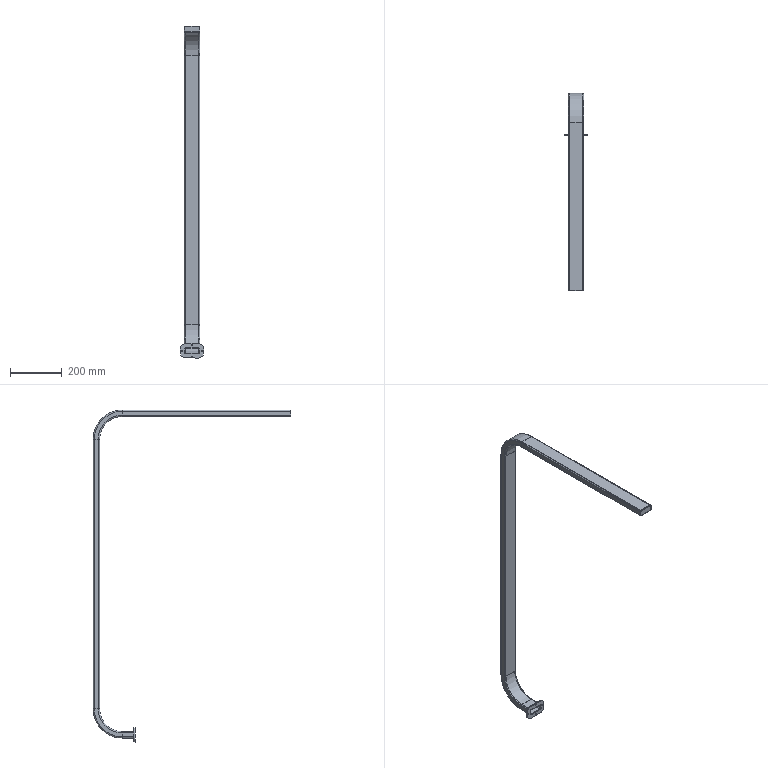Component | SolidWorks | HeightMeasurement-1 | 1 solid | 130 faces | box 90 x 762.5 x 1280 mm | volume 652548 mm3 | cylinder 58 | plane 44 | torus 28 | commonest cylinder face diameters 10 x12 6 x12 5 x8 2 x8 4 x4 40 x4 38.4 x2 225 x2
build123d program:
from build123d import *

# Parameters (mm, degrees)
BOSS_EXTRUDE1_START = -2
BOSS_EXTRUDE1_DEPTH = 2
FILLET1_R           = 2
BOSS_EXTRUDE2_DEPTH = 5
SKETCH6_R           = 2.5
CUT_EXTRUDE1_DEPTH  = 4
CUT_EXTRUDE2_REACH  = 1471.169
SKETCH7_R           = 19.2
FILLET5_R           = 1


with BuildPart() as part:
    # Scan-Thin Part2: sweep along a path in Sketch1
    with BuildLine(Plane(origin=(0, 0, 0), x_dir=(0, 0, -1), z_dir=(1, 0, 0))) as scan_thin_part2_path:
        Line((0, 0), (650, 0))
        ThreePointArc((650, 0), (720.711, -29.289), (750, -100))
        Line((750, -100), (750, -1140))
        ThreePointArc((750, -1140), (720.711, -1210.711), (650, -1240))
        Line((650, -1240), (600, -1240))
    # Sketch3 → Scan-Thin Part2 (sweep)
    with BuildSketch(Plane.XY):
        with BuildLine():
            Line((-25, 12.5), (25, 12.5))
            ThreePointArc((25, 12.5), (28.536, 11.036), (30, 7.5))
            Line((30, 7.5), (30, -7.5))
            ThreePointArc((30, -7.5), (28.536, -11.036), (25, -12.5))
            Line((25, -12.5), (-25, -12.5))
            ThreePointArc((-25, -12.5), (-28.536, -11.036), (-30, -7.5))
            Line((-30, -7.5), (-30, 7.5))
            ThreePointArc((-30, 7.5), (-28.536, 11.036), (-25, 12.5))
        make_face()
        with BuildLine():
            Line((-25, 10.5), (25, 10.5))
            ThreePointArc((25, 10.5), (27.121, 9.621), (28, 7.5))
            Line((28, 7.5), (28, -7.5))
            ThreePointArc((28, -7.5), (27.121, -9.621), (25, -10.5))
            Line((25, -10.5), (-25, -10.5))
            ThreePointArc((-25, -10.5), (-27.121, -9.621), (-28, -7.5))
            Line((-28, -7.5), (-28, 7.5))
            ThreePointArc((-28, 7.5), (-27.121, 9.621), (-25, 10.5))
        make_face(mode=Mode.SUBTRACT)
    sweep(path=scan_thin_part2_path.line)

    # Sketch4 → Boss-Extrude1 (add)
    with BuildSketch(Plane.XY.offset(BOSS_EXTRUDE1_START)):
        with BuildLine():
            Line((28, -7.5), (28, 7.5))
            ThreePointArc((28, 7.5), (27.121, 9.621), (25, 10.5))
            Line((25, 10.5), (-25, 10.5))
            ThreePointArc((-25, 10.5), (-27.121, 9.621), (-28, 7.5))
            Line((-28, 7.5), (-28, -7.5))
            ThreePointArc((-28, -7.5), (-27.121, -9.621), (-25, -10.5))
            Line((-25, -10.5), (25, -10.5))
            ThreePointArc((25, -10.5), (27.121, -9.621), (28, -7.5))
        make_face()
    extrude(amount=BOSS_EXTRUDE1_DEPTH)

    # Fillet1
    fillet1_edges = [part.edges().sort_by_distance(p)[0] for p in [
        (-28.536, -11.036, 0),
        (0, -12.5, 0),
        (28.536, -11.036, 0),
        (30, 0, 0),
        (28.536, 11.036, 0),
        (0, 12.5, 0),
        (-28.536, 11.036, 0),
        (-30, 0, 0),
    ]]
    fillet(fillet1_edges, radius=FILLET1_R)

    # Sketch5 → Boss-Extrude2 (add)
    with BuildSketch(Plane.XY.offset(-600)):
        with BuildLine():
            Line((-25, -1212.5), (25, -1212.5))
            ThreePointArc((25, -1212.5), (39.142, -1218.358), (45, -1232.5))
            Line((45, -1232.5), (45, -1247.5))
            ThreePointArc((45, -1247.5), (39.142, -1261.642), (25, -1267.5))
            Line((25, -1267.5), (-25, -1267.5))
            ThreePointArc((-25, -1267.5), (-39.142, -1261.642), (-45, -1247.5))
            Line((-45, -1247.5), (-45, -1232.5))
            ThreePointArc((-45, -1232.5), (-39.142, -1218.358), (-25, -1212.5))
        make_face()
        with BuildLine():
            Line((-30, -1247.5), (-30, -1232.5))
            ThreePointArc((-30, -1232.5), (-28.536, -1228.964), (-25, -1227.5))
            Line((-25, -1227.5), (25, -1227.5))
            ThreePointArc((25, -1227.5), (28.536, -1228.964), (30, -1232.5))
            Line((30, -1232.5), (30, -1247.5))
            ThreePointArc((30, -1247.5), (28.536, -1251.036), (25, -1252.5))
            Line((25, -1252.5), (-25, -1252.5))
            ThreePointArc((-25, -1252.5), (-28.536, -1251.036), (-30, -1247.5))
        make_face(mode=Mode.SUBTRACT)
    extrude(amount=-BOSS_EXTRUDE2_DEPTH)

    # Sketch6 → Cut-Extrude1 (cut)
    with BuildSketch(Plane.XY.offset(-600)):
        with Locations((0, -1217.5)):
            Circle(SKETCH6_R)
        with Locations((40, -1240)):
            Circle(SKETCH6_R)
        with Locations((0, -1262.5)):
            Circle(SKETCH6_R)
        with Locations((-40, -1240)):
            Circle(SKETCH6_R)
    extrude(amount=-CUT_EXTRUDE1_DEPTH, mode=Mode.SUBTRACT)

    # Sketch7 → Cut-Extrude2 (cut, up to next)
    with BuildSketch(Plane.XZ.offset(12.5), mode=Mode.PRIVATE) as cut_extrude2_sk1:
        with Locations(Location((0, -100, 0), (0, 0, 270))):
            Circle(SKETCH7_R)
    cut_extrude2_tool1 = extrude(cut_extrude2_sk1.sketch, amount=-CUT_EXTRUDE2_REACH, mode=Mode.PRIVATE) & part.part
    add(cut_extrude2_tool1.solids().sort_by_distance((0, -12.5, -100))[0], mode=Mode.SUBTRACT)

    # Fillet5
    fillet5_edges = [part.edges().sort_by_distance(p)[0] for p in [
        (0, -1227.5, -605),
        (-28.536, -1228.964, -605),
        (-30, -1240, -605),
        (-28.536, -1251.036, -605),
        (0, -1252.5, -605),
        (28.536, -1251.036, -605),
        (30, -1240, -605),
        (28.536, -1228.964, -605),
        (-28, -1240, -600),
        (-27.121, -1230.379, -600),
        (0, -1229.5, -600),
        (27.121, -1230.379, -600),
        (28, -1240, -600),
        (27.121, -1249.621, -600),
        (0, -1250.5, -600),
        (-27.121, -1249.621, -600),
    ]]
    fillet(fillet5_edges, radius=FILLET5_R)


solid = part.part

# Placed as in the assembly
solid = solid.moved(Location((1132.686, 963.312, 3448.954), (90, 0, 0)))